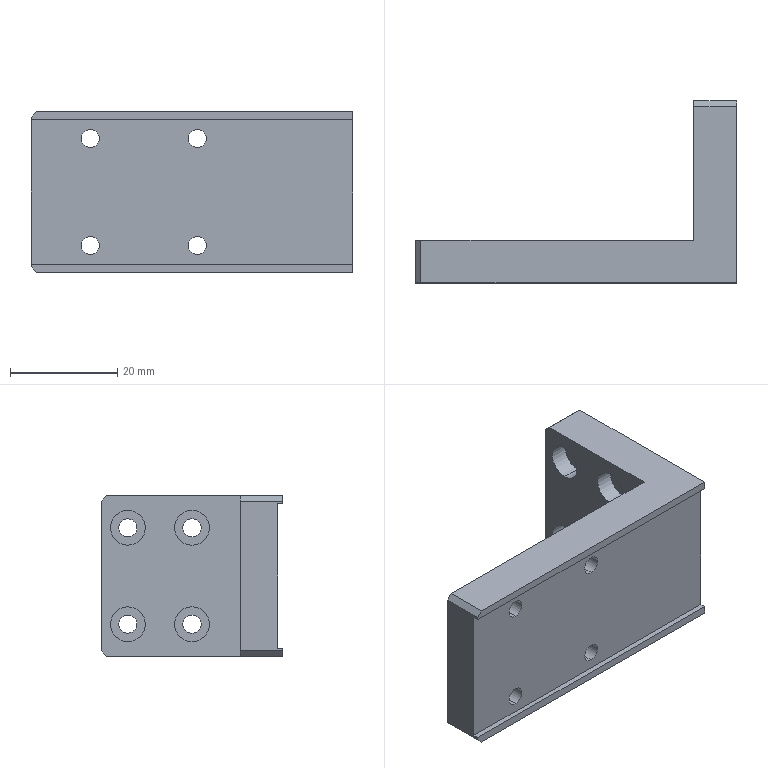Component | SolidWorks | 31298011300CylinderMountingPlate-2 | 1 solid | 64 faces | box 60 x 34 x 30 mm | volume 17601 mm3 | cylinder 36 | plane 24 | cone 4 | commonest cylinder face diameters 3.4 x16 6.5 x16 3.3 x4 | material Q235-A
build123d program:
from build123d import *

# Parameters (mm, degrees)
EXTRUDE_THIN1_DEPTH                             = 15
M3_HEX_SOCKET_HEAD_CAP_SCREW_CBORE1_D           = 3.4
M3_HEX_SOCKET_HEAD_CAP_SCREW_CBORE1_CBORE_D     = 6.5
M3_HEX_SOCKET_HEAD_CAP_SCREW_CBORE1_CBORE_DEPTH = 3.4
LPATTERN1_COUNT                                 = 2
LPATTERN1_PITCH                                 = 20
LPATTERN1_COUNT_DIR2                            = 2
LPATTERN1_PITCH_DIR2                            = 20
M3_HEX_SOCKET_HEAD_CAP_SCREW_CBORE2_D           = 3.4
M3_HEX_SOCKET_HEAD_CAP_SCREW_CBORE2_CBORE_D     = 6.5
M3_HEX_SOCKET_HEAD_CAP_SCREW_CBORE2_CBORE_DEPTH = 3.4
LPATTERN2_COUNT                                 = 2
LPATTERN2_PITCH                                 = 18
LPATTERN2_COUNT_DIR2                            = 2
LPATTERN2_PITCH_DIR2                            = 12
CHAMFER2_SIZE                                   = 1
M4_TAPPED_HOLE3_D                               = 3.3
M4_TAPPED_HOLE3_DEPTH                           = 11.5
M4_TAPPED_HOLE3_TIP                             = 0.9914
SKETCH15_W                                      = 60
SKETCH15_H                                      = 27
CUT_EXTRUDE1_DEPTH                              = 1


with BuildPart() as part:
    # Sketch1 → Extrude-Thin1 (new, symmetric)
    with BuildSketch(Plane.XY):
        Polygon((60, 0), (0, 0), (0, 34), (8, 34), (8, 8), (60, 8), align=None)
    extrude(amount=EXTRUDE_THIN1_DEPTH, both=True)

    # M3 Hex Socket Head Cap Screw CBORE1 (through all)
    with Locations(Plane(origin=(0, 8, 0), x_dir=(-1, 0, 0), z_dir=(0, 1, 0))):
        with Locations((-49, -10)):
            m3_hex_socket_head_cap_screw_cbore1 = CounterBoreHole(M3_HEX_SOCKET_HEAD_CAP_SCREW_CBORE1_D / 2, M3_HEX_SOCKET_HEAD_CAP_SCREW_CBORE1_CBORE_D / 2, M3_HEX_SOCKET_HEAD_CAP_SCREW_CBORE1_CBORE_DEPTH)

    # LPattern1: M3 Hex Socket Head Cap Screw CBORE1 2 × 2
    with Locations(*[(-j * LPATTERN1_PITCH_DIR2, 0, i * LPATTERN1_PITCH) for i in range(LPATTERN1_COUNT) for j in range(LPATTERN1_COUNT_DIR2) if (i, j) != (0, 0)]):
        add(m3_hex_socket_head_cap_screw_cbore1, mode=Mode.SUBTRACT)

    # M3 Hex Socket Head Cap Screw CBORE2 (through all)
    with Locations(Plane(origin=(8, 8.266, -0.21), x_dir=(0, 0, 1), z_dir=(1, 0, 0))):
        with Locations((-8.79, -20.734)):
            m3_hex_socket_head_cap_screw_cbore2 = CounterBoreHole(M3_HEX_SOCKET_HEAD_CAP_SCREW_CBORE2_D / 2, M3_HEX_SOCKET_HEAD_CAP_SCREW_CBORE2_CBORE_D / 2, M3_HEX_SOCKET_HEAD_CAP_SCREW_CBORE2_CBORE_DEPTH)

    # LPattern2: M3 Hex Socket Head Cap Screw CBORE2 2 × 2
    with Locations(*[(0, -j * LPATTERN2_PITCH_DIR2, i * LPATTERN2_PITCH) for i in range(LPATTERN2_COUNT) for j in range(LPATTERN2_COUNT_DIR2) if (i, j) != (0, 0)]):
        add(m3_hex_socket_head_cap_screw_cbore2, mode=Mode.SUBTRACT)

    # Chamfer2
    chamfer2_edges = [part.edges().sort_by_distance(p)[0] for p in [
        (4, 34, -15),
        (4, 34, 15),
        (60, 4, 15),
        (60, 4, -15),
    ]]
    chamfer(chamfer2_edges, length=CHAMFER2_SIZE)

    # M4 Tapped Hole3
    with Locations(Plane.ZY):
        with Locations((-7.5, 6), (7.5, 6)):
            Hole(M4_TAPPED_HOLE3_D / 2, depth=M4_TAPPED_HOLE3_DEPTH)
            with Locations((0, 0, -(M4_TAPPED_HOLE3_DEPTH + M4_TAPPED_HOLE3_TIP / 2))):  # 118° drill point
                Cone(0, M4_TAPPED_HOLE3_D / 2, M4_TAPPED_HOLE3_TIP, mode=Mode.SUBTRACT)

    # Sketch15 → Cut-Extrude1 (cut)
    with BuildSketch(Plane.XZ):
        with Locations((30, 0)):
            Rectangle(SKETCH15_W, SKETCH15_H)
    extrude(amount=-CUT_EXTRUDE1_DEPTH, mode=Mode.SUBTRACT)


solid = part.part

# Placed as in the assembly
solid = solid.moved(Location((143.77, 20.768, 38.329), (-180, 0, 180)))